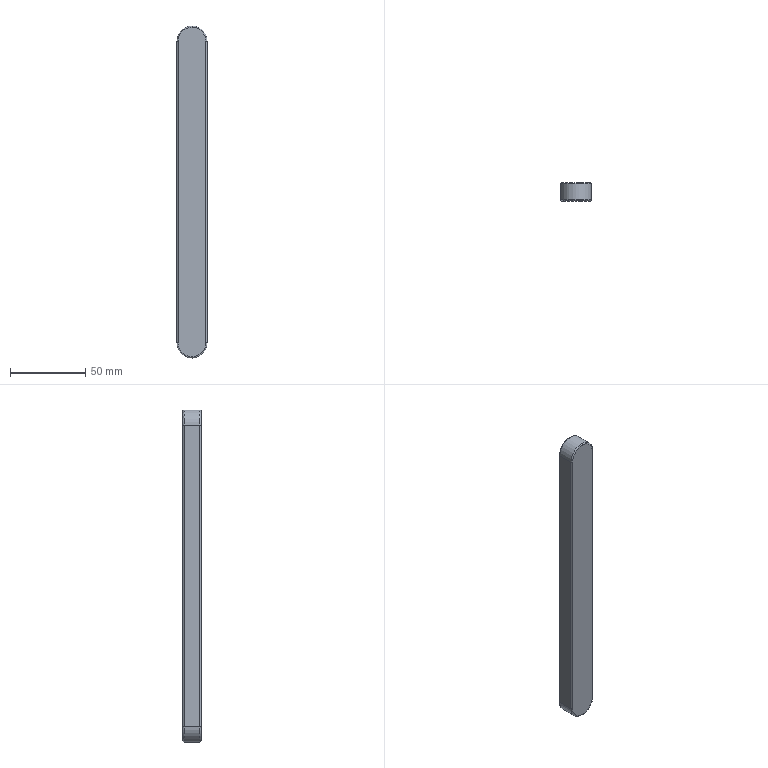Component | SolidWorks | ParallelKey20_220_12-1 | 1 solid | 17 faces | box 20 x 12 x 220 mm | volume 51645 mm3 | cylinder 7 | spline 6 | plane 4 | commonest cylinder face diameters 1.6 x4 20 x3
STEP:
#1=CARTESIAN_POINT('',(8.268,10.394,4.35));
#2=VERTEX_POINT('',#1);
#3=CARTESIAN_POINT('',(8.63,10.394,3.988));
#4=VERTEX_POINT('',#3);
#5=CARTESIAN_POINT('',(8.268,10.394,4.35));
#6=CARTESIAN_POINT('',(8.279,10.394,4.35));
#7=CARTESIAN_POINT('',(8.295,10.394,4.35));
#8=CARTESIAN_POINT('',(8.315,10.394,4.347));
#9=CARTESIAN_POINT('',(8.324,10.394,4.346));
#10=CARTESIAN_POINT('',(8.328,10.394,4.345));
#11=CARTESIAN_POINT('',(8.331,10.394,4.345));
#12=CARTESIAN_POINT('',(8.332,10.394,4.345));
#13=CARTESIAN_POINT('',(8.345,10.394,4.342));
#14=CARTESIAN_POINT('',(8.362,10.394,4.338));
#15=CARTESIAN_POINT('',(8.382,10.394,4.332));
#16=CARTESIAN_POINT('',(8.391,10.394,4.329));
#17=CARTESIAN_POINT('',(8.396,10.394,4.327));
#18=CARTESIAN_POINT('',(8.398,10.394,4.326));
#19=CARTESIAN_POINT('',(8.4,10.394,4.326));
#20=CARTESIAN_POINT('',(8.412,10.394,4.32));
#21=CARTESIAN_POINT('',(8.429,10.394,4.313));
#22=CARTESIAN_POINT('',(8.448,10.394,4.303));
#23=CARTESIAN_POINT('',(8.456,10.394,4.298));
#24=CARTESIAN_POINT('',(8.461,10.394,4.295));
#25=CARTESIAN_POINT('',(8.463,10.394,4.293));
#26=CARTESIAN_POINT('',(8.487,10.394,4.278));
#27=CARTESIAN_POINT('',(8.506,10.394,4.262));
#28=CARTESIAN_POINT('',(8.533,10.394,4.235));
#29=CARTESIAN_POINT('',(8.545,10.394,4.222));
#30=CARTESIAN_POINT('',(8.558,10.394,4.204));
#31=CARTESIAN_POINT('',(8.564,10.394,4.197));
#32=CARTESIAN_POINT('',(8.567,10.394,4.192));
#33=CARTESIAN_POINT('',(8.569,10.394,4.189));
#34=CARTESIAN_POINT('',(8.578,10.394,4.176));
#35=CARTESIAN_POINT('',(8.587,10.394,4.16));
#36=CARTESIAN_POINT('',(8.596,10.394,4.141));
#37=CARTESIAN_POINT('',(8.6,10.394,4.131));
#38=CARTESIAN_POINT('',(8.602,10.394,4.127));
#39=CARTESIAN_POINT('',(8.603,10.394,4.124));
#40=CARTESIAN_POINT('',(8.604,10.394,4.123));
#41=CARTESIAN_POINT('',(8.609,10.394,4.111));
#42=CARTESIAN_POINT('',(8.614,10.394,4.094));
#43=CARTESIAN_POINT('',(8.62,10.394,4.074));
#44=CARTESIAN_POINT('',(8.622,10.394,4.064));
#45=CARTESIAN_POINT('',(8.623,10.394,4.06));
#46=CARTESIAN_POINT('',(8.623,10.394,4.057));
#47=CARTESIAN_POINT('',(8.624,10.394,4.055));
#48=CARTESIAN_POINT('',(8.628,10.394,4.032));
#49=CARTESIAN_POINT('',(8.63,10.394,4.01));
#50=CARTESIAN_POINT('',(8.63,10.394,3.988));
#51=B_SPLINE_CURVE_WITH_KNOTS('',3,(#5,#6,#7,#8,#9,#10,#11,#12,#13,#14,#15,#16,#17,#18,#19,#20,#21,#22,#23,#24,#25,#26,#27,#28,#29,#30,#31,#32,#33,#34,#35,#36,#37,#38,#39,#40,#41,#42,#43,#44,#45,#46,#47,#48,#49,#50),.UNSPECIFIED.,.F.,.F.,(4,1,1,1,2,2,1,1,1,2,2,1,1,2,2,2,1,1,2,2,1,1,1,2,2,1,1,1,2,2,4),(0.,0.0625,0.09375,0.1094,0.1172,0.125,0.1875,0.2187,0.2344,0.2422,0.25,0.3125,0.3437,0.3594,0.375,0.5,0.5625,0.5937,0.6094,0.625,0.6875,0.7187,0.7344,0.7422,0.75,0.8125,0.8437,0.8594,0.8672,0.875,1.),.UNSPECIFIED.);
#52=EDGE_CURVE('',#2,#4,#51,.T.);
#53=ORIENTED_EDGE('',*,*,#52,.F.);
#54=CARTESIAN_POINT('',(8.268,10.362,4.382));
#55=VERTEX_POINT('',#54);
#56=CARTESIAN_POINT('',(8.268,10.362,4.35));
#57=DIRECTION('',(1.,0.,0.));
#58=DIRECTION('',(0.,0.,1.));
#59=AXIS2_PLACEMENT_3D('',#56,#57,#58);
#60=CIRCLE('',#59,0.0315);
#61=EDGE_CURVE('',#2,#55,#60,.T.);
#62=ORIENTED_EDGE('',*,*,#61,.T.);
#63=CARTESIAN_POINT('',(8.661,10.362,3.988));
#64=VERTEX_POINT('',#63);
#65=CARTESIAN_POINT('',(8.268,10.362,3.988));
#66=DIRECTION('',(0.,1.,0.));
#67=DIRECTION('',(0.,0.,1.));
#68=AXIS2_PLACEMENT_3D('',#65,#66,#67);
#69=CIRCLE('',#68,0.3937);
#70=EDGE_CURVE('',#55,#64,#69,.T.);
#71=ORIENTED_EDGE('',*,*,#70,.T.);
#72=CARTESIAN_POINT('',(8.63,10.362,3.988));
#73=DIRECTION('',(-0.,0.,-1.));
#74=DIRECTION('',(1.,0.,0.));
#75=AXIS2_PLACEMENT_3D('',#72,#73,#74);
#76=CIRCLE('',#75,0.0315);
#77=EDGE_CURVE('',#4,#64,#76,.T.);
#78=ORIENTED_EDGE('',*,*,#77,.F.);
#79=EDGE_LOOP('',(#53,#62,#71,#78));
#80=FACE_OUTER_BOUND('',#79,.T.);
#81=CARTESIAN_POINT('',(8.268,10.394,4.35));
#82=CARTESIAN_POINT('',(8.48,10.394,4.35));
#83=CARTESIAN_POINT('',(8.63,10.394,4.2));
#84=CARTESIAN_POINT('',(8.63,10.394,3.988));
#85=CARTESIAN_POINT('',(8.268,10.394,4.369));
#86=CARTESIAN_POINT('',(8.491,10.394,4.369));
#87=CARTESIAN_POINT('',(8.648,10.394,4.211));
#88=CARTESIAN_POINT('',(8.648,10.394,3.988));
#89=CARTESIAN_POINT('',(8.268,10.381,4.382));
#90=CARTESIAN_POINT('',(8.498,10.381,4.382));
#91=CARTESIAN_POINT('',(8.661,10.381,4.219));
#92=CARTESIAN_POINT('',(8.661,10.381,3.988));
#93=CARTESIAN_POINT('',(8.268,10.362,4.382));
#94=CARTESIAN_POINT('',(8.498,10.362,4.382));
#95=CARTESIAN_POINT('',(8.661,10.362,4.219));
#96=CARTESIAN_POINT('',(8.661,10.362,3.988));
#97=(BOUNDED_SURFACE()B_SPLINE_SURFACE(3,3,((#81,#82,#83,#84),(#85,#86,#87,#88),(#89,#90,#91,#92),(#93,#94,#95,#96)),.UNSPECIFIED.,.F.,.F.,.T.)B_SPLINE_SURFACE_WITH_KNOTS((4,4),(4,4),(0.,1.),(0.,1.),.UNSPECIFIED.)GEOMETRIC_REPRESENTATION_ITEM()RATIONAL_B_SPLINE_SURFACE(((1.,0.8047,0.8047,1.),(0.8047,0.6476,0.6476,0.8047),(0.8047,0.6476,0.6476,0.8047),(1.,0.8047,0.8047,1.)))REPRESENTATION_ITEM('')SURFACE());
#98=ADVANCED_FACE('',(#80),#97,.T.);
#99=CARTESIAN_POINT('',(8.268,9.953,4.382));
#100=VERTEX_POINT('',#99);
#101=CARTESIAN_POINT('',(8.661,9.953,3.988));
#102=VERTEX_POINT('',#101);
#103=CARTESIAN_POINT('',(8.268,9.953,3.988));
#104=DIRECTION('',(0.,1.,0.));
#105=DIRECTION('',(0.,0.,-1.));
#106=AXIS2_PLACEMENT_3D('',#103,#104,#105);
#107=CIRCLE('',#106,0.3937);
#108=EDGE_CURVE('',#100,#102,#107,.T.);
#109=ORIENTED_EDGE('',*,*,#108,.F.);
#110=CARTESIAN_POINT('',(8.268,9.921,4.35));
#111=VERTEX_POINT('',#110);
#112=CARTESIAN_POINT('',(8.268,9.953,4.35));
#113=DIRECTION('',(1.,0.,0.));
#114=DIRECTION('',(0.,0.,1.));
#115=AXIS2_PLACEMENT_3D('',#112,#113,#114);
#116=CIRCLE('',#115,0.0315);
#117=EDGE_CURVE('',#100,#111,#116,.T.);
#118=ORIENTED_EDGE('',*,*,#117,.T.);
#119=CARTESIAN_POINT('',(8.63,9.921,3.988));
#120=VERTEX_POINT('',#119);
#121=CARTESIAN_POINT('',(8.268,9.921,4.35));
#122=CARTESIAN_POINT('',(8.48,9.921,4.35));
#123=CARTESIAN_POINT('',(8.63,9.921,4.2));
#124=CARTESIAN_POINT('',(8.63,9.921,3.988));
#125=(BOUNDED_CURVE()B_SPLINE_CURVE(3,(#121,#122,#123,#124),.UNSPECIFIED.,.F.,.F.)B_SPLINE_CURVE_WITH_KNOTS((4,4),(0.,1.),.UNSPECIFIED.)CURVE()GEOMETRIC_REPRESENTATION_ITEM()RATIONAL_B_SPLINE_CURVE((1.,0.8047,0.8047,1.))REPRESENTATION_ITEM(''));
#126=EDGE_CURVE('',#111,#120,#125,.T.);
#127=ORIENTED_EDGE('',*,*,#126,.T.);
#128=CARTESIAN_POINT('',(8.63,9.953,3.988));
#129=DIRECTION('',(-0.,0.,-1.));
#130=DIRECTION('',(-1.,0.,0.));
#131=AXIS2_PLACEMENT_3D('',#128,#129,#130);
#132=CIRCLE('',#131,0.0315);
#133=EDGE_CURVE('',#102,#120,#132,.T.);
#134=ORIENTED_EDGE('',*,*,#133,.F.);
#135=EDGE_LOOP('',(#109,#118,#127,#134));
#136=FACE_OUTER_BOUND('',#135,.T.);
#137=CARTESIAN_POINT('',(8.268,9.953,4.382));
#138=CARTESIAN_POINT('',(8.498,9.953,4.382));
#139=CARTESIAN_POINT('',(8.661,9.953,4.219));
#140=CARTESIAN_POINT('',(8.661,9.953,3.988));
#141=CARTESIAN_POINT('',(8.268,9.934,4.382));
#142=CARTESIAN_POINT('',(8.498,9.934,4.382));
#143=CARTESIAN_POINT('',(8.661,9.934,4.219));
#144=CARTESIAN_POINT('',(8.661,9.934,3.988));
#145=CARTESIAN_POINT('',(8.268,9.921,4.369));
#146=CARTESIAN_POINT('',(8.491,9.921,4.369));
#147=CARTESIAN_POINT('',(8.648,9.921,4.211));
#148=CARTESIAN_POINT('',(8.648,9.921,3.988));
#149=CARTESIAN_POINT('',(8.268,9.921,4.35));
#150=CARTESIAN_POINT('',(8.48,9.921,4.35));
#151=CARTESIAN_POINT('',(8.63,9.921,4.2));
#152=CARTESIAN_POINT('',(8.63,9.921,3.988));
#153=(BOUNDED_SURFACE()B_SPLINE_SURFACE(3,3,((#137,#138,#139,#140),(#141,#142,#143,#144),(#145,#146,#147,#148),(#149,#150,#151,#152)),.UNSPECIFIED.,.F.,.F.,.T.)B_SPLINE_SURFACE_WITH_KNOTS((4,4),(4,4),(0.,1.),(0.,1.),.UNSPECIFIED.)GEOMETRIC_REPRESENTATION_ITEM()RATIONAL_B_SPLINE_SURFACE(((1.,0.8047,0.8047,1.),(0.8047,0.6476,0.6476,0.8047),(0.8047,0.6476,0.6476,0.8047),(1.,0.8047,0.8047,1.)))REPRESENTATION_ITEM('')SURFACE());
#154=ADVANCED_FACE('',(#136),#153,.T.);
#155=CARTESIAN_POINT('',(8.268,10.362,-4.28));
#156=VERTEX_POINT('',#155);
#157=CARTESIAN_POINT('',(7.874,10.362,-3.886));
#158=VERTEX_POINT('',#157);
#159=CARTESIAN_POINT('',(8.268,10.362,-3.886));
#160=DIRECTION('',(0.,1.,0.));
#161=DIRECTION('',(0.,0.,1.));
#162=AXIS2_PLACEMENT_3D('',#159,#160,#161);
#163=CIRCLE('',#162,0.3937);
#164=EDGE_CURVE('',#156,#158,#163,.T.);
#165=ORIENTED_EDGE('',*,*,#164,.F.);
#166=CARTESIAN_POINT('',(8.268,9.953,-4.28));
#167=VERTEX_POINT('',#166);
#168=CARTESIAN_POINT('',(8.268,10.394,-4.28));
#169=DIRECTION('',(0.,-1.,0.));
#170=VECTOR('',#169,39.37);
#171=LINE('',#168,#170);
#172=EDGE_CURVE('',#156,#167,#171,.T.);
#173=ORIENTED_EDGE('',*,*,#172,.T.);
#174=CARTESIAN_POINT('',(7.874,9.953,-3.886));
#175=VERTEX_POINT('',#174);
#176=CARTESIAN_POINT('',(8.268,9.953,-3.886));
#177=DIRECTION('',(0.,1.,0.));
#178=DIRECTION('',(0.,0.,-1.));
#179=AXIS2_PLACEMENT_3D('',#176,#177,#178);
#180=CIRCLE('',#179,0.3937);
#181=EDGE_CURVE('',#167,#175,#180,.T.);
#182=ORIENTED_EDGE('',*,*,#181,.T.);
#183=CARTESIAN_POINT('',(7.874,10.394,-3.886));
#184=DIRECTION('',(0.,1.,0.));
#185=VECTOR('',#184,39.37);
#186=LINE('',#183,#185);
#187=EDGE_CURVE('',#175,#158,#186,.T.);
#188=ORIENTED_EDGE('',*,*,#187,.T.);
#189=EDGE_LOOP('',(#165,#173,#182,#188));
#190=FACE_OUTER_BOUND('',#189,.T.);
#191=CARTESIAN_POINT('',(8.268,10.394,-3.886));
#192=DIRECTION('',(0.,-1.,0.));
#193=DIRECTION('',(0.,0.,-1.));
#194=AXIS2_PLACEMENT_3D('',#191,#192,#193);
#195=CYLINDRICAL_SURFACE('',#194,0.3937);
#196=ADVANCED_FACE('',(#190),#195,.T.);
#197=CARTESIAN_POINT('',(8.63,10.394,-3.886));
#198=VERTEX_POINT('',#197);
#199=CARTESIAN_POINT('',(8.63,10.394,-3.886));
#200=DIRECTION('',(0.,0.,-1.));
#201=VECTOR('',#200,39.37);
#202=LINE('',#199,#201);
#203=EDGE_CURVE('',#4,#198,#202,.T.);
#204=ORIENTED_EDGE('',*,*,#203,.T.);
#205=CARTESIAN_POINT('',(7.906,10.394,-3.886));
#206=VERTEX_POINT('',#205);
#207=CARTESIAN_POINT('',(8.63,10.394,-3.886));
#208=CARTESIAN_POINT('',(8.63,10.394,-3.897));
#209=CARTESIAN_POINT('',(8.629,10.394,-3.913));
#210=CARTESIAN_POINT('',(8.627,10.394,-3.933));
#211=CARTESIAN_POINT('',(8.626,10.394,-3.942));
#212=CARTESIAN_POINT('',(8.625,10.394,-3.946));
#213=CARTESIAN_POINT('',(8.624,10.394,-3.949));
#214=CARTESIAN_POINT('',(8.624,10.394,-3.95));
#215=CARTESIAN_POINT('',(8.622,10.394,-3.963));
#216=CARTESIAN_POINT('',(8.618,10.394,-3.98));
#217=CARTESIAN_POINT('',(8.612,10.394,-4.));
#218=CARTESIAN_POINT('',(8.608,10.394,-4.01));
#219=CARTESIAN_POINT('',(8.607,10.394,-4.014));
#220=CARTESIAN_POINT('',(8.606,10.394,-4.016));
#221=CARTESIAN_POINT('',(8.605,10.394,-4.018));
#222=CARTESIAN_POINT('',(8.6,10.394,-4.031));
#223=CARTESIAN_POINT('',(8.592,10.394,-4.047));
#224=CARTESIAN_POINT('',(8.582,10.394,-4.066));
#225=CARTESIAN_POINT('',(8.577,10.394,-4.074));
#226=CARTESIAN_POINT('',(8.574,10.394,-4.079));
#227=CARTESIAN_POINT('',(8.573,10.394,-4.081));
#228=CARTESIAN_POINT('',(8.557,10.394,-4.105));
#229=CARTESIAN_POINT('',(8.542,10.394,-4.124));
#230=CARTESIAN_POINT('',(8.515,10.394,-4.151));
#231=CARTESIAN_POINT('',(8.501,10.394,-4.163));
#232=CARTESIAN_POINT('',(8.484,10.394,-4.177));
#233=CARTESIAN_POINT('',(8.476,10.394,-4.182));
#234=CARTESIAN_POINT('',(8.471,10.394,-4.186));
#235=CARTESIAN_POINT('',(8.468,10.394,-4.187));
#236=CARTESIAN_POINT('',(8.456,10.394,-4.196));
#237=CARTESIAN_POINT('',(8.44,10.394,-4.205));
#238=CARTESIAN_POINT('',(8.421,10.394,-4.214));
#239=CARTESIAN_POINT('',(8.411,10.394,-4.219));
#240=CARTESIAN_POINT('',(8.407,10.394,-4.22));
#241=CARTESIAN_POINT('',(8.404,10.394,-4.221));
#242=CARTESIAN_POINT('',(8.402,10.394,-4.222));
#243=CARTESIAN_POINT('',(8.39,10.394,-4.227));
#244=CARTESIAN_POINT('',(8.374,10.394,-4.233));
#245=CARTESIAN_POINT('',(8.354,10.394,-4.238));
#246=CARTESIAN_POINT('',(8.344,10.394,-4.24));
#247=CARTESIAN_POINT('',(8.339,10.394,-4.241));
#248=CARTESIAN_POINT('',(8.337,10.394,-4.241));
#249=CARTESIAN_POINT('',(8.335,10.394,-4.242));
#250=CARTESIAN_POINT('',(8.312,10.394,-4.246));
#251=CARTESIAN_POINT('',(8.29,10.394,-4.248));
#252=CARTESIAN_POINT('',(8.257,10.394,-4.248));
#253=CARTESIAN_POINT('',(8.24,10.394,-4.247));
#254=CARTESIAN_POINT('',(8.221,10.394,-4.245));
#255=CARTESIAN_POINT('',(8.211,10.394,-4.244));
#256=CARTESIAN_POINT('',(8.207,10.394,-4.243));
#257=CARTESIAN_POINT('',(8.205,10.394,-4.242));
#258=CARTESIAN_POINT('',(8.203,10.394,-4.242));
#259=CARTESIAN_POINT('',(8.19,10.394,-4.24));
#260=CARTESIAN_POINT('',(8.173,10.394,-4.236));
#261=CARTESIAN_POINT('',(8.154,10.394,-4.23));
#262=CARTESIAN_POINT('',(8.144,10.394,-4.226));
#263=CARTESIAN_POINT('',(8.14,10.394,-4.225));
#264=CARTESIAN_POINT('',(8.137,10.394,-4.224));
#265=CARTESIAN_POINT('',(8.136,10.394,-4.223));
#266=CARTESIAN_POINT('',(8.123,10.394,-4.218));
#267=CARTESIAN_POINT('',(8.106,10.394,-4.211));
#268=CARTESIAN_POINT('',(8.088,10.394,-4.2));
#269=CARTESIAN_POINT('',(8.08,10.394,-4.196));
#270=CARTESIAN_POINT('',(8.075,10.394,-4.192));
#271=CARTESIAN_POINT('',(8.072,10.394,-4.191));
#272=CARTESIAN_POINT('',(8.049,10.394,-4.175));
#273=CARTESIAN_POINT('',(8.029,10.394,-4.16));
#274=CARTESIAN_POINT('',(8.003,10.394,-4.133));
#275=CARTESIAN_POINT('',(7.99,10.394,-4.119));
#276=CARTESIAN_POINT('',(7.977,10.394,-4.102));
#277=CARTESIAN_POINT('',(7.972,10.394,-4.094));
#278=CARTESIAN_POINT('',(7.968,10.394,-4.089));
#279=CARTESIAN_POINT('',(7.966,10.394,-4.087));
#280=CARTESIAN_POINT('',(7.958,10.394,-4.074));
#281=CARTESIAN_POINT('',(7.949,10.394,-4.058));
#282=CARTESIAN_POINT('',(7.939,10.394,-4.039));
#283=CARTESIAN_POINT('',(7.935,10.394,-4.029));
#284=CARTESIAN_POINT('',(7.933,10.394,-4.025));
#285=CARTESIAN_POINT('',(7.932,10.394,-4.022));
#286=CARTESIAN_POINT('',(7.931,10.394,-4.021));
#287=CARTESIAN_POINT('',(7.927,10.394,-4.008));
#288=CARTESIAN_POINT('',(7.921,10.394,-3.992));
#289=CARTESIAN_POINT('',(7.916,10.394,-3.972));
#290=CARTESIAN_POINT('',(7.914,10.394,-3.962));
#291=CARTESIAN_POINT('',(7.913,10.394,-3.958));
#292=CARTESIAN_POINT('',(7.912,10.394,-3.955));
#293=CARTESIAN_POINT('',(7.912,10.394,-3.953));
#294=CARTESIAN_POINT('',(7.908,10.394,-3.93));
#295=CARTESIAN_POINT('',(7.906,10.394,-3.908));
#296=CARTESIAN_POINT('',(7.906,10.394,-3.886));
#297=B_SPLINE_CURVE_WITH_KNOTS('',3,(#207,#208,#209,#210,#211,#212,#213,#214,#215,#216,#217,#218,#219,#220,#221,#222,#223,#224,#225,#226,#227,#228,#229,#230,#231,#232,#233,#234,#235,#236,#237,#238,#239,#240,#241,#242,#243,#244,#245,#246,#247,#248,#249,#250,#251,#252,#253,#254,#255,#256,#257,#258,#259,#260,#261,#262,#263,#264,#265,#266,#267,#268,#269,#270,#271,#272,#273,#274,#275,#276,#277,#278,#279,#280,#281,#282,#283,#284,#285,#286,#287,#288,#289,#290,#291,#292,#293,#294,#295,#296),.UNSPECIFIED.,.F.,.F.,(4,1,1,1,2,2,1,1,1,2,2,1,1,2,2,2,1,1,2,2,1,1,1,2,2,1,1,1,2,2,2,1,1,1,2,2,1,1,1,2,2,1,1,2,2,2,1,1,2,2,1,1,1,2,2,1,1,1,2,2,4),(0.,0.03125,0.04688,0.05469,0.05859,0.0625,0.09375,0.1094,0.1172,0.1211,0.125,0.1563,0.1719,0.1797,0.1875,0.25,0.2813,0.2969,0.3047,0.3125,0.3438,0.3594,0.3672,0.3711,0.375,0.4063,0.4219,0.4297,0.4336,0.4375,0.5,0.5313,0.5469,0.5547,0.5586,0.5625,0.5938,0.6094,0.6172,0.6211,0.625,0.6563,0.6719,0.6797,0.6875,0.75,0.7813,0.7969,0.8047,0.8125,0.8438,0.8594,0.8672,0.8711,0.875,0.9063,0.9219,0.9297,0.9336,0.9375,1.),.UNSPECIFIED.);
#298=EDGE_CURVE('',#198,#206,#297,.T.);
#299=ORIENTED_EDGE('',*,*,#298,.T.);
#300=CARTESIAN_POINT('',(7.906,10.394,3.988));
#301=VERTEX_POINT('',#300);
#302=CARTESIAN_POINT('',(7.906,10.394,-3.886));
#303=DIRECTION('',(-0.,0.,1.));
#304=VECTOR('',#303,39.37);
#305=LINE('',#302,#304);
#306=EDGE_CURVE('',#206,#301,#305,.T.);
#307=ORIENTED_EDGE('',*,*,#306,.T.);
#308=CARTESIAN_POINT('',(7.906,10.394,3.988));
#309=CARTESIAN_POINT('',(7.906,10.394,3.999));
#310=CARTESIAN_POINT('',(7.906,10.394,4.016));
#311=CARTESIAN_POINT('',(7.908,10.394,4.035));
#312=CARTESIAN_POINT('',(7.91,10.394,4.045));
#313=CARTESIAN_POINT('',(7.911,10.394,4.049));
#314=CARTESIAN_POINT('',(7.911,10.394,4.051));
#315=CARTESIAN_POINT('',(7.911,10.394,4.053));
#316=CARTESIAN_POINT('',(7.914,10.394,4.066));
#317=CARTESIAN_POINT('',(7.918,10.394,4.083));
#318=CARTESIAN_POINT('',(7.924,10.394,4.102));
#319=CARTESIAN_POINT('',(7.927,10.394,4.112));
#320=CARTESIAN_POINT('',(7.929,10.394,4.116));
#321=CARTESIAN_POINT('',(7.93,10.394,4.119));
#322=CARTESIAN_POINT('',(7.93,10.394,4.12));
#323=CARTESIAN_POINT('',(7.935,10.394,4.133));
#324=CARTESIAN_POINT('',(7.943,10.394,4.15));
#325=CARTESIAN_POINT('',(7.953,10.394,4.168));
#326=CARTESIAN_POINT('',(7.958,10.394,4.176));
#327=CARTESIAN_POINT('',(7.961,10.394,4.181));
#328=CARTESIAN_POINT('',(7.963,10.394,4.184));
#329=CARTESIAN_POINT('',(7.978,10.394,4.207));
#330=CARTESIAN_POINT('',(7.994,10.394,4.227));
#331=CARTESIAN_POINT('',(8.02,10.394,4.253));
#332=CARTESIAN_POINT('',(8.034,10.394,4.266));
#333=CARTESIAN_POINT('',(8.052,10.394,4.279));
#334=CARTESIAN_POINT('',(8.059,10.394,4.284));
#335=CARTESIAN_POINT('',(8.064,10.394,4.288));
#336=CARTESIAN_POINT('',(8.067,10.394,4.29));
#337=CARTESIAN_POINT('',(8.08,10.394,4.298));
#338=CARTESIAN_POINT('',(8.096,10.394,4.307));
#339=CARTESIAN_POINT('',(8.115,10.394,4.317));
#340=CARTESIAN_POINT('',(8.124,10.394,4.321));
#341=CARTESIAN_POINT('',(8.129,10.394,4.323));
#342=CARTESIAN_POINT('',(8.132,10.394,4.324));
#343=CARTESIAN_POINT('',(8.133,10.394,4.324));
#344=CARTESIAN_POINT('',(8.145,10.394,4.329));
#345=CARTESIAN_POINT('',(8.162,10.394,4.335));
#346=CARTESIAN_POINT('',(8.182,10.394,4.34));
#347=CARTESIAN_POINT('',(8.192,10.394,4.342));
#348=CARTESIAN_POINT('',(8.196,10.394,4.343));
#349=CARTESIAN_POINT('',(8.199,10.394,4.344));
#350=CARTESIAN_POINT('',(8.2,10.394,4.344));
#351=CARTESIAN_POINT('',(8.224,10.394,4.348));
#352=CARTESIAN_POINT('',(8.246,10.394,4.35));
#353=CARTESIAN_POINT('',(8.268,10.394,4.35));
#354=B_SPLINE_CURVE_WITH_KNOTS('',3,(#308,#309,#310,#311,#312,#313,#314,#315,#316,#317,#318,#319,#320,#321,#322,#323,#324,#325,#326,#327,#328,#329,#330,#331,#332,#333,#334,#335,#336,#337,#338,#339,#340,#341,#342,#343,#344,#345,#346,#347,#348,#349,#350,#351,#352,#353),.UNSPECIFIED.,.F.,.F.,(4,1,1,1,2,2,1,1,1,2,2,1,1,2,2,2,1,1,2,2,1,1,1,2,2,1,1,1,2,2,4),(0.,0.0625,0.09375,0.1094,0.1172,0.125,0.1875,0.2187,0.2344,0.2422,0.25,0.3125,0.3437,0.3594,0.375,0.5,0.5625,0.5937,0.6094,0.625,0.6875,0.7187,0.7344,0.7422,0.75,0.8125,0.8437,0.8594,0.8672,0.875,1.),.UNSPECIFIED.);
#355=EDGE_CURVE('',#301,#2,#354,.T.);
#356=ORIENTED_EDGE('',*,*,#355,.T.);
#357=ORIENTED_EDGE('',*,*,#52,.T.);
#358=EDGE_LOOP('',(#204,#299,#307,#356,#357));
#359=FACE_OUTER_BOUND('',#358,.T.);
#360=CARTESIAN_POINT('',(8.268,10.394,-3.886));
#361=DIRECTION('',(0.,1.,0.));
#362=DIRECTION('',(-0.,0.,1.));
#363=AXIS2_PLACEMENT_3D('',#360,#361,#362);
#364=PLANE('',#363);
#365=ADVANCED_FACE('',(#359),#364,.T.);
#366=CARTESIAN_POINT('',(7.906,10.362,-3.886));
#367=DIRECTION('',(0.,0.,-1.));
#368=DIRECTION('',(-1.,0.,0.));
#369=AXIS2_PLACEMENT_3D('',#366,#367,#368);
#370=CIRCLE('',#369,0.0315);
#371=EDGE_CURVE('',#158,#206,#370,.T.);
#372=ORIENTED_EDGE('',*,*,#371,.T.);
#373=ORIENTED_EDGE('',*,*,#298,.F.);
#374=CARTESIAN_POINT('',(8.661,10.362,-3.886));
#375=VERTEX_POINT('',#374);
#376=CARTESIAN_POINT('',(8.63,10.362,-3.886));
#377=DIRECTION('',(0.,0.,-1.));
#378=DIRECTION('',(1.,0.,0.));
#379=AXIS2_PLACEMENT_3D('',#376,#377,#378);
#380=CIRCLE('',#379,0.0315);
#381=EDGE_CURVE('',#198,#375,#380,.T.);
#382=ORIENTED_EDGE('',*,*,#381,.T.);
#383=CARTESIAN_POINT('',(8.268,10.362,-3.886));
#384=DIRECTION('',(0.,1.,0.));
#385=DIRECTION('',(0.,0.,1.));
#386=AXIS2_PLACEMENT_3D('',#383,#384,#385);
#387=CIRCLE('',#386,0.3937);
#388=EDGE_CURVE('',#375,#156,#387,.T.);
#389=ORIENTED_EDGE('',*,*,#388,.T.);
#390=ORIENTED_EDGE('',*,*,#164,.T.);
#391=EDGE_LOOP('',(#372,#373,#382,#389,#390));
#392=FACE_OUTER_BOUND('',#391,.T.);
#393=CARTESIAN_POINT('',(8.63,10.394,-3.886));
#394=CARTESIAN_POINT('',(8.63,10.394,-4.61));
#395=CARTESIAN_POINT('',(7.906,10.394,-4.61));
#396=CARTESIAN_POINT('',(7.906,10.394,-3.886));
#397=CARTESIAN_POINT('',(8.648,10.394,-3.886));
#398=CARTESIAN_POINT('',(8.648,10.394,-4.647));
#399=CARTESIAN_POINT('',(7.887,10.394,-4.647));
#400=CARTESIAN_POINT('',(7.887,10.394,-3.886));
#401=CARTESIAN_POINT('',(8.661,10.381,-3.886));
#402=CARTESIAN_POINT('',(8.661,10.381,-4.673));
#403=CARTESIAN_POINT('',(7.874,10.381,-4.673));
#404=CARTESIAN_POINT('',(7.874,10.381,-3.886));
#405=CARTESIAN_POINT('',(8.661,10.362,-3.886));
#406=CARTESIAN_POINT('',(8.661,10.362,-4.673));
#407=CARTESIAN_POINT('',(7.874,10.362,-4.673));
#408=CARTESIAN_POINT('',(7.874,10.362,-3.886));
#409=(BOUNDED_SURFACE()B_SPLINE_SURFACE(3,3,((#393,#394,#395,#396),(#397,#398,#399,#400),(#401,#402,#403,#404),(#405,#406,#407,#408)),.UNSPECIFIED.,.F.,.F.,.T.)B_SPLINE_SURFACE_WITH_KNOTS((4,4),(4,4),(0.,1.),(0.,1.),.UNSPECIFIED.)GEOMETRIC_REPRESENTATION_ITEM()RATIONAL_B_SPLINE_SURFACE(((1.,0.3333,0.3333,1.),(0.8047,0.2682,0.2682,0.8047),(0.8047,0.2682,0.2682,0.8047),(1.,0.3333,0.3333,1.)))REPRESENTATION_ITEM('')SURFACE());
#410=ADVANCED_FACE('',(#392),#409,.T.);
#411=ORIENTED_EDGE('',*,*,#77,.T.);
#412=CARTESIAN_POINT('',(8.661,10.362,-3.886));
#413=DIRECTION('',(-0.,0.,-1.));
#414=VECTOR('',#413,39.37);
#415=LINE('',#412,#414);
#416=EDGE_CURVE('',#64,#375,#415,.T.);
#417=ORIENTED_EDGE('',*,*,#416,.T.);
#418=ORIENTED_EDGE('',*,*,#381,.F.);
#419=ORIENTED_EDGE('',*,*,#203,.F.);
#420=EDGE_LOOP('',(#411,#417,#418,#419));
#421=FACE_OUTER_BOUND('',#420,.T.);
#422=CARTESIAN_POINT('',(8.63,10.362,-3.886));
#423=DIRECTION('',(0.,0.,1.));
#424=DIRECTION('',(1.,0.,0.));
#425=AXIS2_PLACEMENT_3D('',#422,#423,#424);
#426=CYLINDRICAL_SURFACE('',#425,0.0315);
#427=ADVANCED_FACE('',(#421),#426,.T.);
#428=ORIENTED_EDGE('',*,*,#61,.F.);
#429=ORIENTED_EDGE('',*,*,#355,.F.);
#430=CARTESIAN_POINT('',(7.874,10.362,3.988));
#431=VERTEX_POINT('',#430);
#432=CARTESIAN_POINT('',(7.906,10.362,3.988));
#433=DIRECTION('',(-0.,0.,1.));
#434=DIRECTION('',(-1.,0.,0.));
#435=AXIS2_PLACEMENT_3D('',#432,#433,#434);
#436=CIRCLE('',#435,0.0315);
#437=EDGE_CURVE('',#301,#431,#436,.T.);
#438=ORIENTED_EDGE('',*,*,#437,.T.);
#439=CARTESIAN_POINT('',(8.268,10.362,3.988));
#440=DIRECTION('',(0.,1.,0.));
#441=DIRECTION('',(0.,0.,1.));
#442=AXIS2_PLACEMENT_3D('',#439,#440,#441);
#443=CIRCLE('',#442,0.3937);
#444=EDGE_CURVE('',#431,#55,#443,.T.);
#445=ORIENTED_EDGE('',*,*,#444,.T.);
#446=EDGE_LOOP('',(#428,#429,#438,#445));
#447=FACE_OUTER_BOUND('',#446,.T.);
#448=CARTESIAN_POINT('',(7.906,10.394,3.988));
#449=CARTESIAN_POINT('',(7.906,10.394,4.2));
#450=CARTESIAN_POINT('',(8.056,10.394,4.35));
#451=CARTESIAN_POINT('',(8.268,10.394,4.35));
#452=CARTESIAN_POINT('',(7.887,10.394,3.988));
#453=CARTESIAN_POINT('',(7.887,10.394,4.211));
#454=CARTESIAN_POINT('',(8.045,10.394,4.369));
#455=CARTESIAN_POINT('',(8.268,10.394,4.369));
#456=CARTESIAN_POINT('',(7.874,10.381,3.988));
#457=CARTESIAN_POINT('',(7.874,10.381,4.219));
#458=CARTESIAN_POINT('',(8.037,10.381,4.382));
#459=CARTESIAN_POINT('',(8.268,10.381,4.382));
#460=CARTESIAN_POINT('',(7.874,10.362,3.988));
#461=CARTESIAN_POINT('',(7.874,10.362,4.219));
#462=CARTESIAN_POINT('',(8.037,10.362,4.382));
#463=CARTESIAN_POINT('',(8.268,10.362,4.382));
#464=(BOUNDED_SURFACE()B_SPLINE_SURFACE(3,3,((#448,#449,#450,#451),(#452,#453,#454,#455),(#456,#457,#458,#459),(#460,#461,#462,#463)),.UNSPECIFIED.,.F.,.F.,.T.)B_SPLINE_SURFACE_WITH_KNOTS((4,4),(4,4),(0.,1.),(0.,1.),.UNSPECIFIED.)GEOMETRIC_REPRESENTATION_ITEM()RATIONAL_B_SPLINE_SURFACE(((1.,0.8047,0.8047,1.),(0.8047,0.6476,0.6476,0.8047),(0.8047,0.6476,0.6476,0.8047),(1.,0.8047,0.8047,1.)))REPRESENTATION_ITEM('')SURFACE());
#465=ADVANCED_FACE('',(#447),#464,.T.);
#466=ORIENTED_EDGE('',*,*,#437,.F.);
#467=ORIENTED_EDGE('',*,*,#306,.F.);
#468=ORIENTED_EDGE('',*,*,#371,.F.);
#469=CARTESIAN_POINT('',(7.874,10.362,-3.886));
#470=DIRECTION('',(-0.,0.,1.));
#471=VECTOR('',#470,39.37);
#472=LINE('',#469,#471);
#473=EDGE_CURVE('',#158,#431,#472,.T.);
#474=ORIENTED_EDGE('',*,*,#473,.T.);
#475=EDGE_LOOP('',(#466,#467,#468,#474));
#476=FACE_OUTER_BOUND('',#475,.T.);
#477=CARTESIAN_POINT('',(7.906,10.362,-3.886));
#478=DIRECTION('',(0.,0.,-1.));
#479=DIRECTION('',(-1.,0.,0.));
#480=AXIS2_PLACEMENT_3D('',#477,#478,#479);
#481=CYLINDRICAL_SURFACE('',#480,0.0315);
#482=ADVANCED_FACE('',(#476),#481,.T.);
#483=ORIENTED_EDGE('',*,*,#172,.F.);
#484=ORIENTED_EDGE('',*,*,#388,.F.);
#485=CARTESIAN_POINT('',(8.661,9.953,-3.886));
#486=VERTEX_POINT('',#485);
#487=CARTESIAN_POINT('',(8.661,10.394,-3.886));
#488=DIRECTION('',(0.,-1.,0.));
#489=VECTOR('',#488,39.37);
#490=LINE('',#487,#489);
#491=EDGE_CURVE('',#375,#486,#490,.T.);
#492=ORIENTED_EDGE('',*,*,#491,.T.);
#493=CARTESIAN_POINT('',(8.268,9.953,-3.886));
#494=DIRECTION('',(0.,1.,0.));
#495=DIRECTION('',(0.,0.,-1.));
#496=AXIS2_PLACEMENT_3D('',#493,#494,#495);
#497=CIRCLE('',#496,0.3937);
#498=EDGE_CURVE('',#486,#167,#497,.T.);
#499=ORIENTED_EDGE('',*,*,#498,.T.);
#500=EDGE_LOOP('',(#483,#484,#492,#499));
#501=FACE_OUTER_BOUND('',#500,.T.);
#502=CARTESIAN_POINT('',(8.268,10.394,-3.886));
#503=DIRECTION('',(0.,-1.,0.));
#504=DIRECTION('',(0.,0.,-1.));
#505=AXIS2_PLACEMENT_3D('',#502,#503,#504);
#506=CYLINDRICAL_SURFACE('',#505,0.3937);
#507=ADVANCED_FACE('',(#501),#506,.T.);
#508=ORIENTED_EDGE('',*,*,#416,.F.);
#509=CARTESIAN_POINT('',(8.661,10.394,3.988));
#510=DIRECTION('',(0.,1.,0.));
#511=VECTOR('',#510,39.37);
#512=LINE('',#509,#511);
#513=EDGE_CURVE('',#102,#64,#512,.T.);
#514=ORIENTED_EDGE('',*,*,#513,.F.);
#515=CARTESIAN_POINT('',(8.661,9.953,-3.886));
#516=DIRECTION('',(0.,0.,1.));
#517=VECTOR('',#516,39.37);
#518=LINE('',#515,#517);
#519=EDGE_CURVE('',#486,#102,#518,.T.);
#520=ORIENTED_EDGE('',*,*,#519,.F.);
#521=ORIENTED_EDGE('',*,*,#491,.F.);
#522=EDGE_LOOP('',(#508,#514,#520,#521));
#523=FACE_OUTER_BOUND('',#522,.T.);
#524=CARTESIAN_POINT('',(8.661,10.394,-3.886));
#525=DIRECTION('',(-1.,0.,0.));
#526=DIRECTION('',(0.,0.,1.));
#527=AXIS2_PLACEMENT_3D('',#524,#525,#526);
#528=PLANE('',#527);
#529=ADVANCED_FACE('',(#523),#528,.F.);
#530=CARTESIAN_POINT('',(7.874,9.953,3.988));
#531=VERTEX_POINT('',#530);
#532=CARTESIAN_POINT('',(7.874,10.394,3.988));
#533=DIRECTION('',(0.,-1.,0.));
#534=VECTOR('',#533,39.37);
#535=LINE('',#532,#534);
#536=EDGE_CURVE('',#431,#531,#535,.T.);
#537=ORIENTED_EDGE('',*,*,#536,.T.);
#538=CARTESIAN_POINT('',(8.268,9.953,3.988));
#539=DIRECTION('',(0.,1.,0.));
#540=DIRECTION('',(0.,0.,-1.));
#541=AXIS2_PLACEMENT_3D('',#538,#539,#540);
#542=CIRCLE('',#541,0.3937);
#543=EDGE_CURVE('',#531,#100,#542,.T.);
#544=ORIENTED_EDGE('',*,*,#543,.T.);
#545=ORIENTED_EDGE('',*,*,#108,.T.);
#546=ORIENTED_EDGE('',*,*,#513,.T.);
#547=ORIENTED_EDGE('',*,*,#70,.F.);
#548=ORIENTED_EDGE('',*,*,#444,.F.);
#549=EDGE_LOOP('',(#537,#544,#545,#546,#547,#548));
#550=FACE_OUTER_BOUND('',#549,.T.);
#551=CARTESIAN_POINT('',(8.268,10.394,3.988));
#552=DIRECTION('',(0.,-1.,0.));
#553=DIRECTION('',(0.,0.,-1.));
#554=AXIS2_PLACEMENT_3D('',#551,#552,#553);
#555=CYLINDRICAL_SURFACE('',#554,0.3937);
#556=ADVANCED_FACE('',(#550),#555,.T.);
#557=ORIENTED_EDGE('',*,*,#473,.F.);
#558=ORIENTED_EDGE('',*,*,#187,.F.);
#559=CARTESIAN_POINT('',(7.874,9.953,-3.886));
#560=DIRECTION('',(0.,0.,-1.));
#561=VECTOR('',#560,39.37);
#562=LINE('',#559,#561);
#563=EDGE_CURVE('',#531,#175,#562,.T.);
#564=ORIENTED_EDGE('',*,*,#563,.F.);
#565=ORIENTED_EDGE('',*,*,#536,.F.);
#566=EDGE_LOOP('',(#557,#558,#564,#565));
#567=FACE_OUTER_BOUND('',#566,.T.);
#568=CARTESIAN_POINT('',(7.874,10.394,-3.886));
#569=DIRECTION('',(1.,0.,0.));
#570=DIRECTION('',(0.,0.,-1.));
#571=AXIS2_PLACEMENT_3D('',#568,#569,#570);
#572=PLANE('',#571);
#573=ADVANCED_FACE('',(#567),#572,.F.);
#574=ORIENTED_EDGE('',*,*,#498,.F.);
#575=CARTESIAN_POINT('',(8.63,9.921,-3.886));
#576=VERTEX_POINT('',#575);
#577=CARTESIAN_POINT('',(8.63,9.953,-3.886));
#578=DIRECTION('',(0.,0.,-1.));
#579=DIRECTION('',(1.,0.,0.));
#580=AXIS2_PLACEMENT_3D('',#577,#578,#579);
#581=CIRCLE('',#580,0.0315);
#582=EDGE_CURVE('',#486,#576,#581,.T.);
#583=ORIENTED_EDGE('',*,*,#582,.T.);
#584=CARTESIAN_POINT('',(7.906,9.921,-3.886));
#585=VERTEX_POINT('',#584);
#586=CARTESIAN_POINT('',(8.63,9.921,-3.886));
#587=CARTESIAN_POINT('',(8.63,9.921,-4.61));
#588=CARTESIAN_POINT('',(7.906,9.921,-4.61));
#589=CARTESIAN_POINT('',(7.906,9.921,-3.886));
#590=(BOUNDED_CURVE()B_SPLINE_CURVE(3,(#586,#587,#588,#589),.UNSPECIFIED.,.F.,.F.)B_SPLINE_CURVE_WITH_KNOTS((4,4),(0.,1.),.UNSPECIFIED.)CURVE()GEOMETRIC_REPRESENTATION_ITEM()RATIONAL_B_SPLINE_CURVE((1.,0.3333,0.3333,1.))REPRESENTATION_ITEM(''));
#591=EDGE_CURVE('',#576,#585,#590,.T.);
#592=ORIENTED_EDGE('',*,*,#591,.T.);
#593=CARTESIAN_POINT('',(7.906,9.953,-3.886));
#594=DIRECTION('',(0.,0.,-1.));
#595=DIRECTION('',(-1.,0.,0.));
#596=AXIS2_PLACEMENT_3D('',#593,#594,#595);
#597=CIRCLE('',#596,0.0315);
#598=EDGE_CURVE('',#585,#175,#597,.T.);
#599=ORIENTED_EDGE('',*,*,#598,.T.);
#600=ORIENTED_EDGE('',*,*,#181,.F.);
#601=EDGE_LOOP('',(#574,#583,#592,#599,#600));
#602=FACE_OUTER_BOUND('',#601,.T.);
#603=CARTESIAN_POINT('',(8.661,9.953,-3.886));
#604=CARTESIAN_POINT('',(8.661,9.953,-4.673));
#605=CARTESIAN_POINT('',(7.874,9.953,-4.673));
#606=CARTESIAN_POINT('',(7.874,9.953,-3.886));
#607=CARTESIAN_POINT('',(8.661,9.934,-3.886));
#608=CARTESIAN_POINT('',(8.661,9.934,-4.673));
#609=CARTESIAN_POINT('',(7.874,9.934,-4.673));
#610=CARTESIAN_POINT('',(7.874,9.934,-3.886));
#611=CARTESIAN_POINT('',(8.648,9.921,-3.886));
#612=CARTESIAN_POINT('',(8.648,9.921,-4.647));
#613=CARTESIAN_POINT('',(7.887,9.921,-4.647));
#614=CARTESIAN_POINT('',(7.887,9.921,-3.886));
#615=CARTESIAN_POINT('',(8.63,9.921,-3.886));
#616=CARTESIAN_POINT('',(8.63,9.921,-4.61));
#617=CARTESIAN_POINT('',(7.906,9.921,-4.61));
#618=CARTESIAN_POINT('',(7.906,9.921,-3.886));
#619=(BOUNDED_SURFACE()B_SPLINE_SURFACE(3,3,((#603,#604,#605,#606),(#607,#608,#609,#610),(#611,#612,#613,#614),(#615,#616,#617,#618)),.UNSPECIFIED.,.F.,.F.,.T.)B_SPLINE_SURFACE_WITH_KNOTS((4,4),(4,4),(0.,1.),(0.,1.),.UNSPECIFIED.)GEOMETRIC_REPRESENTATION_ITEM()RATIONAL_B_SPLINE_SURFACE(((1.,0.3333,0.3333,1.),(0.8047,0.2682,0.2682,0.8047),(0.8047,0.2682,0.2682,0.8047),(1.,0.3333,0.3333,1.)))REPRESENTATION_ITEM('')SURFACE());
#620=ADVANCED_FACE('',(#602),#619,.T.);
#621=ORIENTED_EDGE('',*,*,#133,.T.);
#622=CARTESIAN_POINT('',(8.63,9.921,-3.886));
#623=DIRECTION('',(-0.,0.,-1.));
#624=VECTOR('',#623,39.37);
#625=LINE('',#622,#624);
#626=EDGE_CURVE('',#120,#576,#625,.T.);
#627=ORIENTED_EDGE('',*,*,#626,.T.);
#628=ORIENTED_EDGE('',*,*,#582,.F.);
#629=ORIENTED_EDGE('',*,*,#519,.T.);
#630=EDGE_LOOP('',(#621,#627,#628,#629));
#631=FACE_OUTER_BOUND('',#630,.T.);
#632=CARTESIAN_POINT('',(8.63,9.953,-3.886));
#633=DIRECTION('',(-0.,0.,-1.));
#634=DIRECTION('',(-1.,0.,0.));
#635=AXIS2_PLACEMENT_3D('',#632,#633,#634);
#636=CYLINDRICAL_SURFACE('',#635,0.0315);
#637=ADVANCED_FACE('',(#631),#636,.T.);
#638=ORIENTED_EDGE('',*,*,#117,.F.);
#639=ORIENTED_EDGE('',*,*,#543,.F.);
#640=CARTESIAN_POINT('',(7.906,9.921,3.988));
#641=VERTEX_POINT('',#640);
#642=CARTESIAN_POINT('',(7.906,9.953,3.988));
#643=DIRECTION('',(-0.,0.,1.));
#644=DIRECTION('',(-1.,0.,0.));
#645=AXIS2_PLACEMENT_3D('',#642,#643,#644);
#646=CIRCLE('',#645,0.0315);
#647=EDGE_CURVE('',#531,#641,#646,.T.);
#648=ORIENTED_EDGE('',*,*,#647,.T.);
#649=CARTESIAN_POINT('',(7.906,9.921,3.988));
#650=CARTESIAN_POINT('',(7.906,9.921,4.2));
#651=CARTESIAN_POINT('',(8.056,9.921,4.35));
#652=CARTESIAN_POINT('',(8.268,9.921,4.35));
#653=(BOUNDED_CURVE()B_SPLINE_CURVE(3,(#649,#650,#651,#652),.UNSPECIFIED.,.F.,.T.)B_SPLINE_CURVE_WITH_KNOTS((4,4),(0.,1.),.UNSPECIFIED.)CURVE()GEOMETRIC_REPRESENTATION_ITEM()RATIONAL_B_SPLINE_CURVE((1.,0.8047,0.8047,1.))REPRESENTATION_ITEM(''));
#654=EDGE_CURVE('',#641,#111,#653,.T.);
#655=ORIENTED_EDGE('',*,*,#654,.T.);
#656=EDGE_LOOP('',(#638,#639,#648,#655));
#657=FACE_OUTER_BOUND('',#656,.T.);
#658=CARTESIAN_POINT('',(7.874,9.953,3.988));
#659=CARTESIAN_POINT('',(7.874,9.953,4.219));
#660=CARTESIAN_POINT('',(8.037,9.953,4.382));
#661=CARTESIAN_POINT('',(8.268,9.953,4.382));
#662=CARTESIAN_POINT('',(7.874,9.934,3.988));
#663=CARTESIAN_POINT('',(7.874,9.934,4.219));
#664=CARTESIAN_POINT('',(8.037,9.934,4.382));
#665=CARTESIAN_POINT('',(8.268,9.934,4.382));
#666=CARTESIAN_POINT('',(7.887,9.921,3.988));
#667=CARTESIAN_POINT('',(7.887,9.921,4.211));
#668=CARTESIAN_POINT('',(8.045,9.921,4.369));
#669=CARTESIAN_POINT('',(8.268,9.921,4.369));
#670=CARTESIAN_POINT('',(7.906,9.921,3.988));
#671=CARTESIAN_POINT('',(7.906,9.921,4.2));
#672=CARTESIAN_POINT('',(8.056,9.921,4.35));
#673=CARTESIAN_POINT('',(8.268,9.921,4.35));
#674=(BOUNDED_SURFACE()B_SPLINE_SURFACE(3,3,((#658,#659,#660,#661),(#662,#663,#664,#665),(#666,#667,#668,#669),(#670,#671,#672,#673)),.UNSPECIFIED.,.F.,.F.,.T.)B_SPLINE_SURFACE_WITH_KNOTS((4,4),(4,4),(0.,1.),(0.,1.),.UNSPECIFIED.)GEOMETRIC_REPRESENTATION_ITEM()RATIONAL_B_SPLINE_SURFACE(((1.,0.8047,0.8047,1.),(0.8047,0.6476,0.6476,0.8047),(0.8047,0.6476,0.6476,0.8047),(1.,0.8047,0.8047,1.)))REPRESENTATION_ITEM('')SURFACE());
#675=ADVANCED_FACE('',(#657),#674,.T.);
#676=ORIENTED_EDGE('',*,*,#647,.F.);
#677=ORIENTED_EDGE('',*,*,#563,.T.);
#678=ORIENTED_EDGE('',*,*,#598,.F.);
#679=CARTESIAN_POINT('',(7.906,9.921,-3.886));
#680=DIRECTION('',(-0.,0.,1.));
#681=VECTOR('',#680,39.37);
#682=LINE('',#679,#681);
#683=EDGE_CURVE('',#585,#641,#682,.T.);
#684=ORIENTED_EDGE('',*,*,#683,.T.);
#685=EDGE_LOOP('',(#676,#677,#678,#684));
#686=FACE_OUTER_BOUND('',#685,.T.);
#687=CARTESIAN_POINT('',(7.906,9.953,-3.886));
#688=DIRECTION('',(-0.,0.,1.));
#689=DIRECTION('',(1.,0.,0.));
#690=AXIS2_PLACEMENT_3D('',#687,#688,#689);
#691=CYLINDRICAL_SURFACE('',#690,0.0315);
#692=ADVANCED_FACE('',(#686),#691,.T.);
#693=ORIENTED_EDGE('',*,*,#126,.F.);
#694=ORIENTED_EDGE('',*,*,#654,.F.);
#695=ORIENTED_EDGE('',*,*,#683,.F.);
#696=ORIENTED_EDGE('',*,*,#591,.F.);
#697=ORIENTED_EDGE('',*,*,#626,.F.);
#698=EDGE_LOOP('',(#693,#694,#695,#696,#697));
#699=FACE_OUTER_BOUND('',#698,.T.);
#700=CARTESIAN_POINT('',(8.268,9.921,-3.886));
#701=DIRECTION('',(0.,1.,0.));
#702=DIRECTION('',(-0.,0.,1.));
#703=AXIS2_PLACEMENT_3D('',#700,#701,#702);
#704=PLANE('',#703);
#705=ADVANCED_FACE('',(#699),#704,.F.);
#706=CLOSED_SHELL('',(#98,#154,#196,#365,#410,#427,#465,#482,#507,#529,#556,#573,#620,#637,#675,#692,#705));
#707=MANIFOLD_SOLID_BREP('',#706);
#708=CARTESIAN_POINT('',(0.,0.,0.));
#709=DIRECTION('',(0.,0.,1.));
#710=DIRECTION('',(1.,0.,0.));
#711=AXIS2_PLACEMENT_3D('',#708,#709,#710);
#712=(LENGTH_UNIT()NAMED_UNIT(*)SI_UNIT($,.METRE.));
#713=LENGTH_MEASURE_WITH_UNIT(LENGTH_MEASURE(0.0254),#712);
#714=DIMENSIONAL_EXPONENTS(1.,0.,0.,0.,0.,0.,0.);
#715=(CONVERSION_BASED_UNIT('',#713)LENGTH_UNIT()NAMED_UNIT(#714));
#716=UNCERTAINTY_MEASURE_WITH_UNIT(LENGTH_MEASURE(0.00001),#715,'','');
#717=(NAMED_UNIT(*)PLANE_ANGLE_UNIT()SI_UNIT($,.RADIAN.));
#718=(NAMED_UNIT(*)SI_UNIT($,.STERADIAN.)SOLID_ANGLE_UNIT());
#719=(GEOMETRIC_REPRESENTATION_CONTEXT(3)GLOBAL_UNCERTAINTY_ASSIGNED_CONTEXT((#716))GLOBAL_UNIT_ASSIGNED_CONTEXT((#715,#717,#718))REPRESENTATION_CONTEXT('',''));
#720=ADVANCED_BREP_SHAPE_REPRESENTATION('',(#707,#711),#719);
#721=COLOUR_RGB('',0.7922,0.8196,0.9333);
#722=FILL_AREA_STYLE_COLOUR('',#721);
#723=FILL_AREA_STYLE('',(#722));
#724=SURFACE_STYLE_FILL_AREA(#723);
#725=SURFACE_SIDE_STYLE('',(#724));
#726=SURFACE_STYLE_USAGE(.BOTH.,#725);
#727=PRESENTATION_STYLE_ASSIGNMENT((#726));
#728=STYLED_ITEM('',(#727),#707);
#729=PRESENTATION_LAYER_ASSIGNMENT('','',(#728));
#730=(LENGTH_UNIT()NAMED_UNIT(*)SI_UNIT($,.METRE.));
#731=LENGTH_MEASURE_WITH_UNIT(LENGTH_MEASURE(0.0254),#730);
#732=DIMENSIONAL_EXPONENTS(1.,0.,0.,0.,0.,0.,0.);
#733=(CONVERSION_BASED_UNIT('',#731)LENGTH_UNIT()NAMED_UNIT(#732));
#734=UNCERTAINTY_MEASURE_WITH_UNIT(LENGTH_MEASURE(0.00001),#733,'','');
#735=(NAMED_UNIT(*)PLANE_ANGLE_UNIT()SI_UNIT($,.RADIAN.));
#736=(NAMED_UNIT(*)SI_UNIT($,.STERADIAN.)SOLID_ANGLE_UNIT());
#737=(GEOMETRIC_REPRESENTATION_CONTEXT(3)GLOBAL_UNCERTAINTY_ASSIGNED_CONTEXT((#734))GLOBAL_UNIT_ASSIGNED_CONTEXT((#733,#735,#736))REPRESENTATION_CONTEXT('',''));
#738=MECHANICAL_DESIGN_GEOMETRIC_PRESENTATION_REPRESENTATION('',(#728),#737);